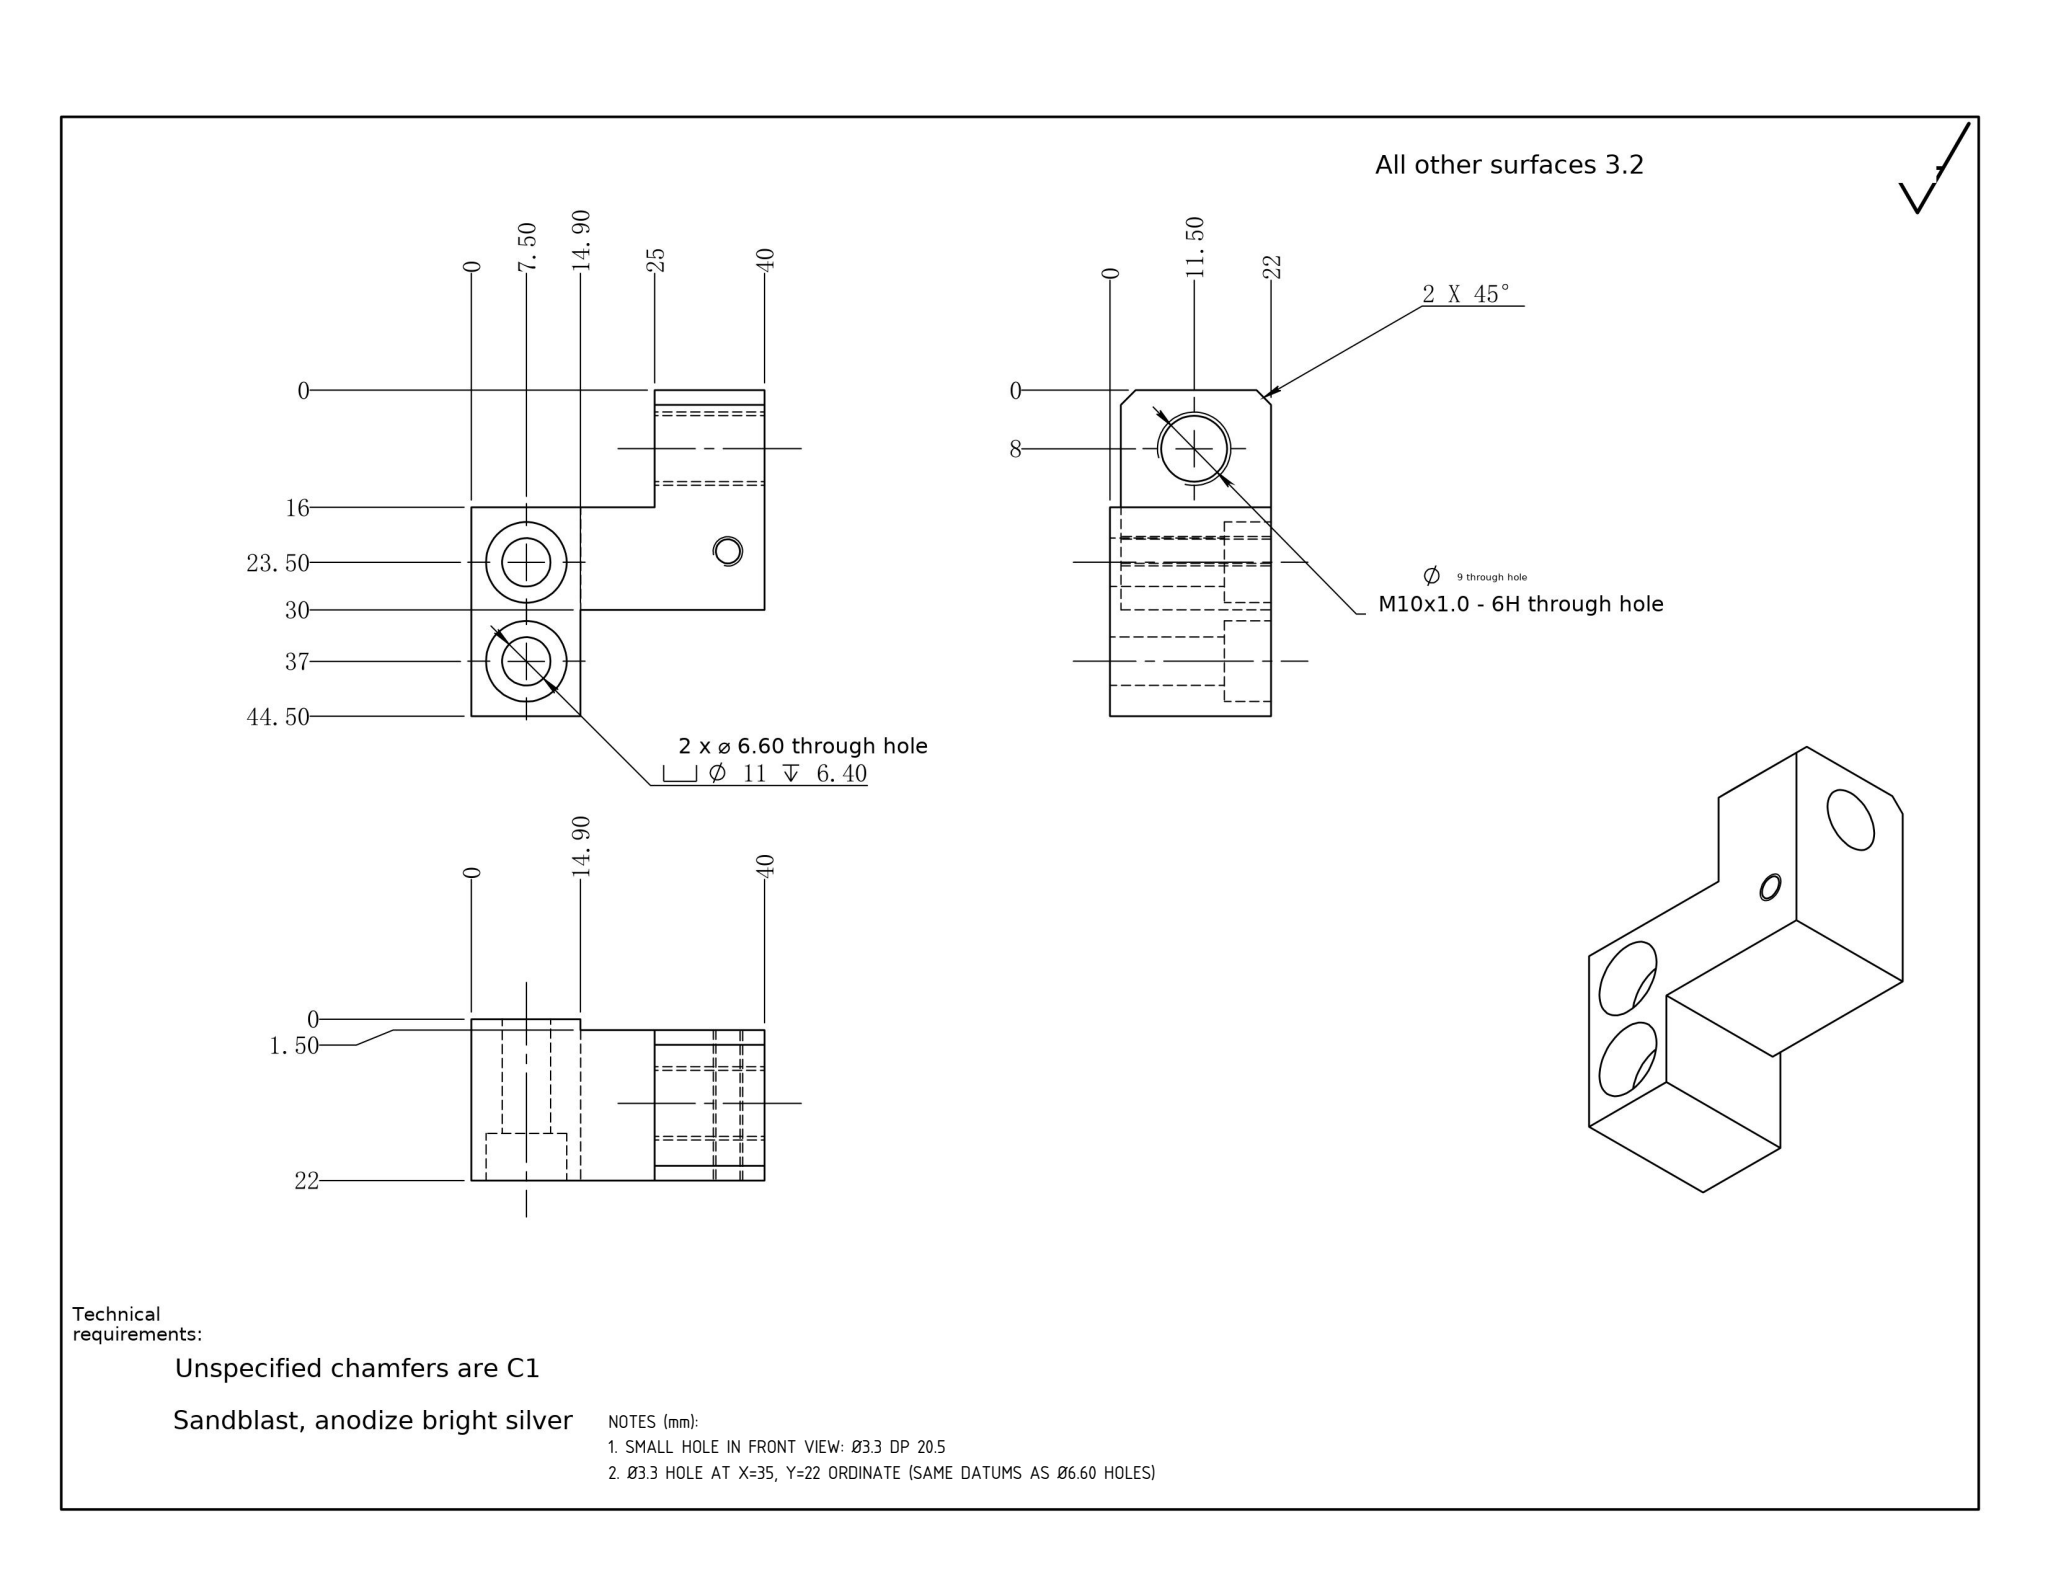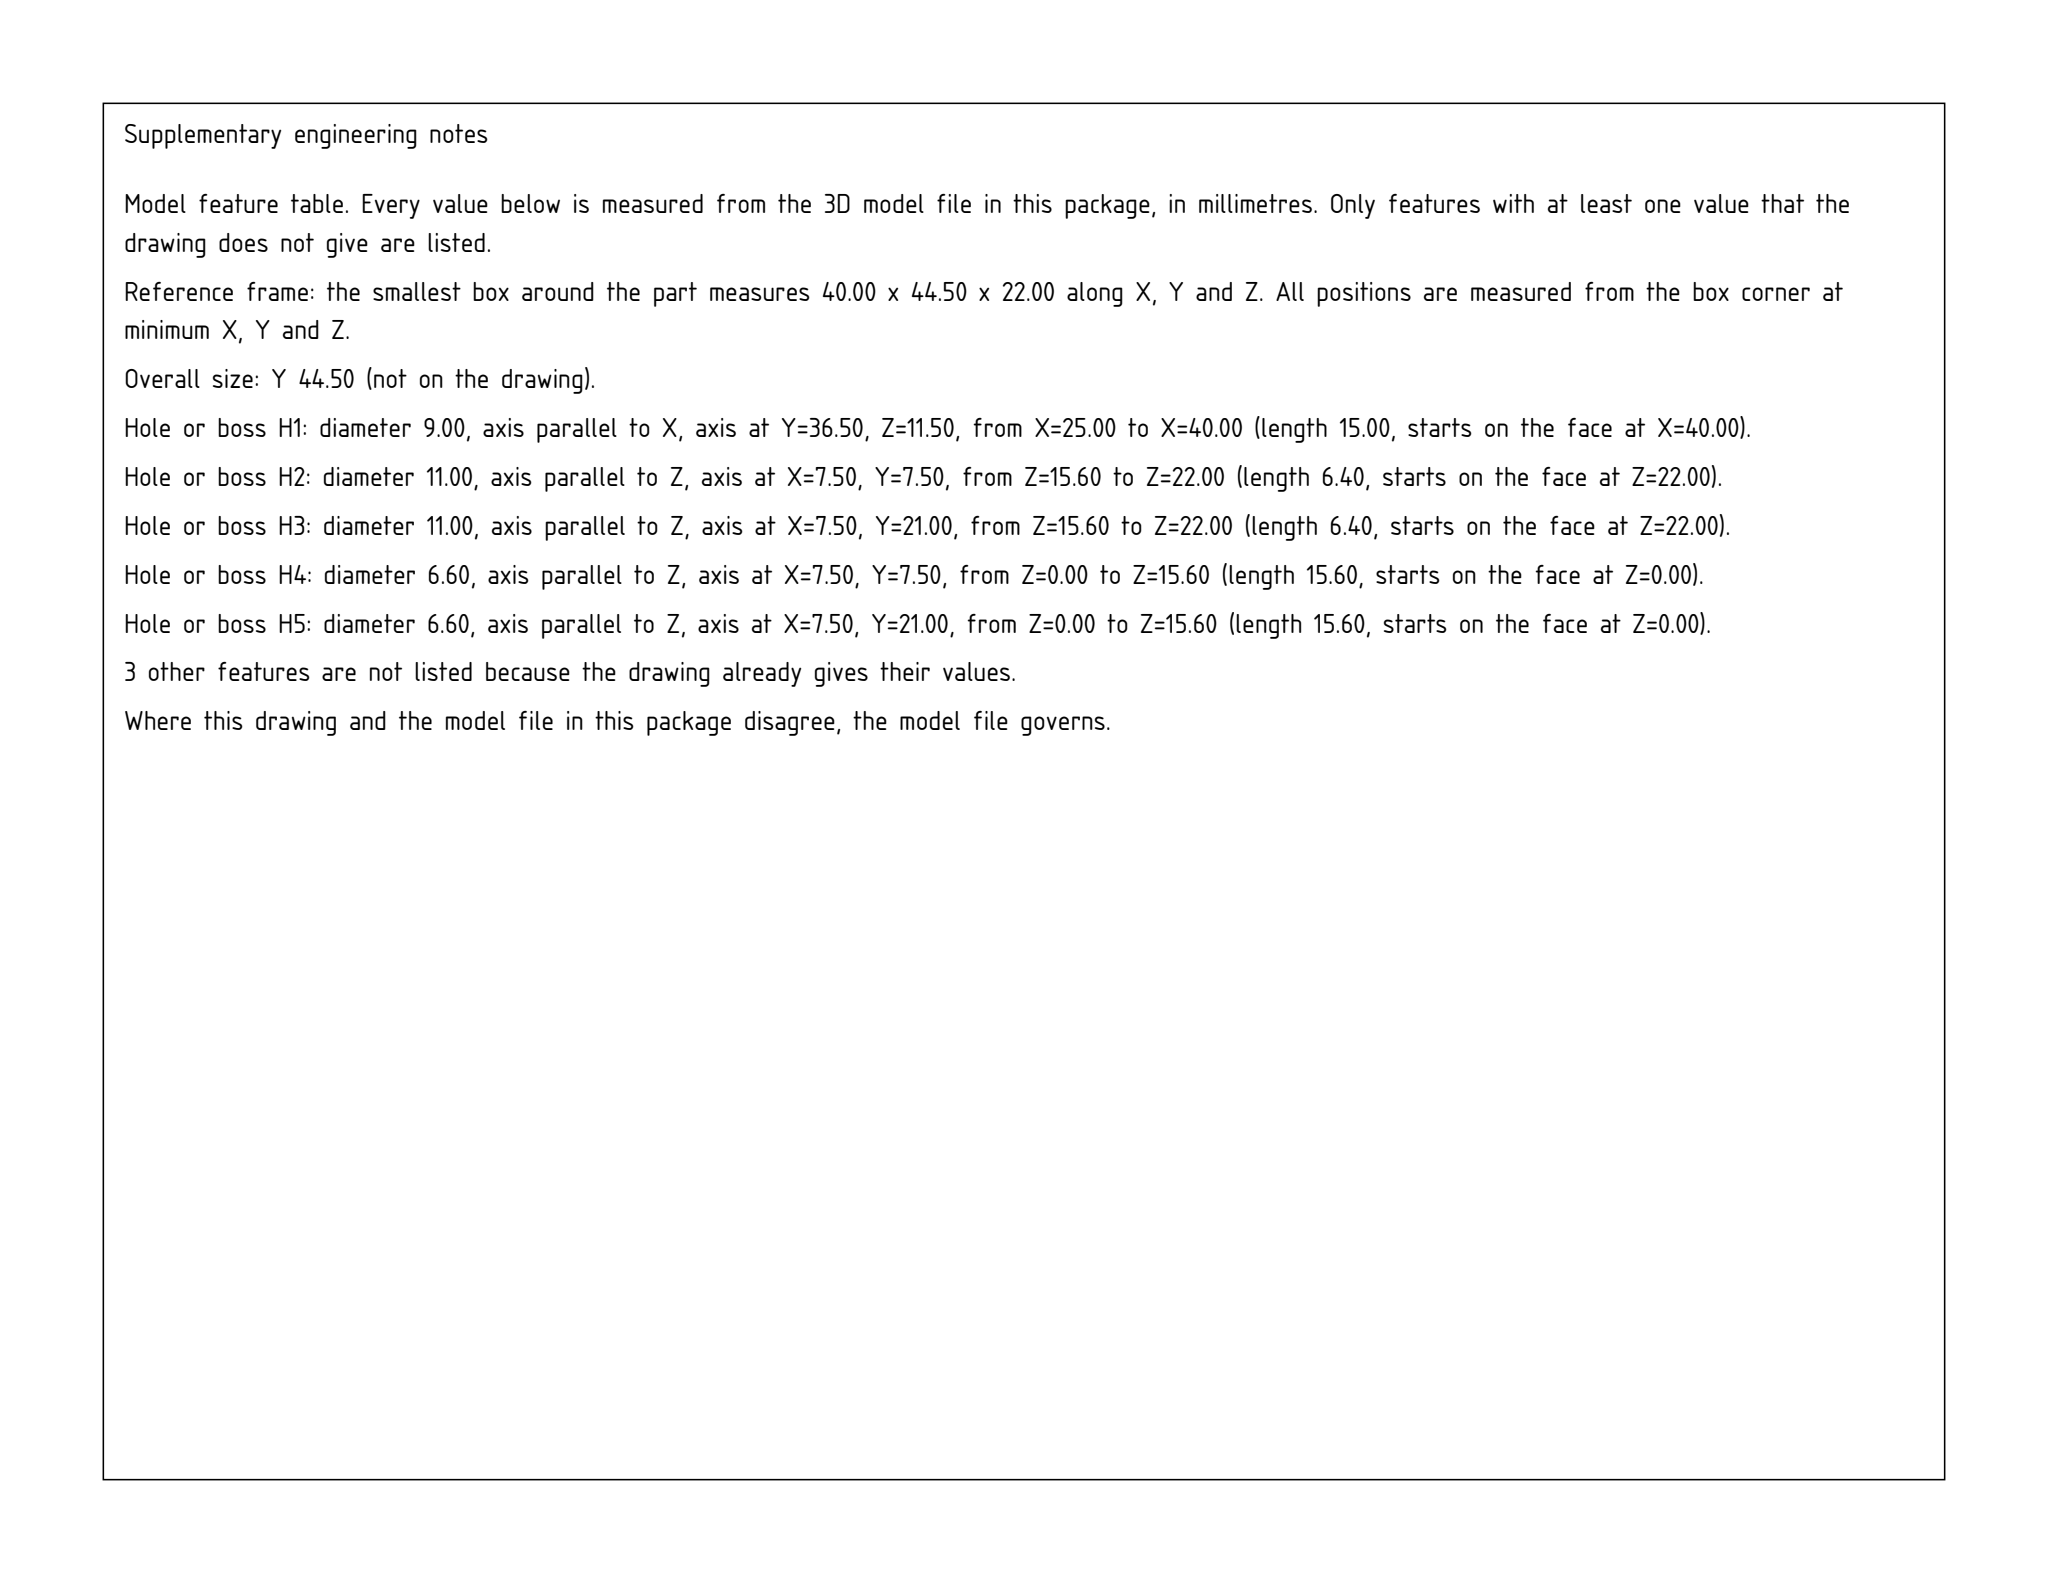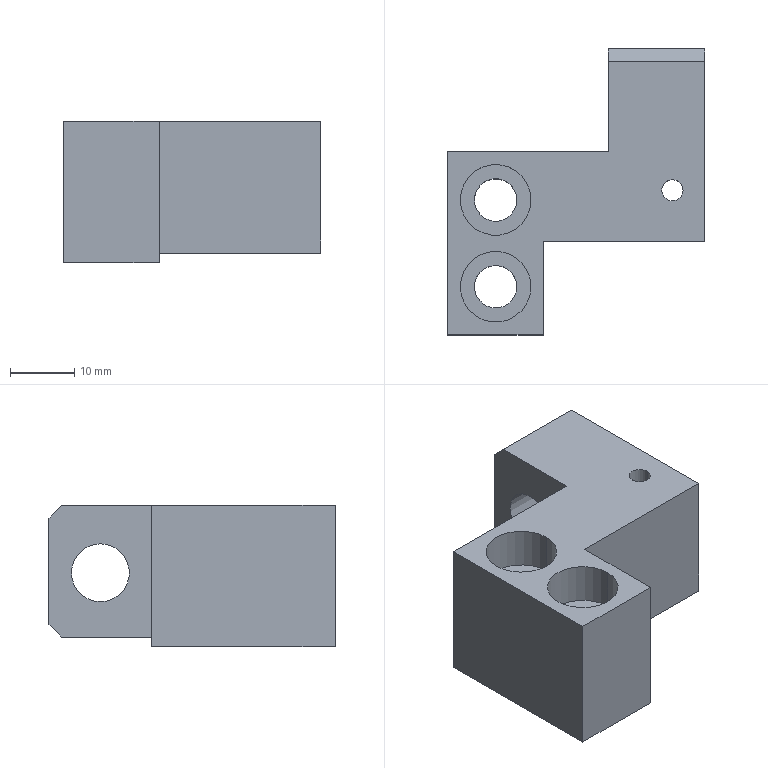Part | SolidWorks | mm | 1 solid | 27 faces | box 40 x 44.5 x 22 mm | volume 17993 mm3 | plane 15 | cylinder 12 | commonest cylinder face diameters 11 x4 6.6 x4 3.3 x2 9 x2
Drawing notes:
SMALL HOLE IN FRONT VIEW: Ø3.3 DP 20.5 | from the solid: cylinder dia 3.3, axis z, length 20.5 (blind, part 22 thick)
Ø3.3 HOLE AT X=35, Y=22 ORDINATE (SAME DATUMS AS Ø6.60 HOLES) | from the solid: pos [35.0, 22.5]; Y ordinate = 44.5-22.5 = 22, matching chain where y=21->23.50, y=7.5->37
build123d program:
from build123d import *

# Parameters (mm, degrees)
SKETCH1_W                                       = 40
SKETCH1_H                                       = 44.5
BOSS_EXTRUDE1_DEPTH                             = 22
M6_HEX_SOCKET_HEAD_CAP_SCREW_CBORE2_D           = 6.6
M6_HEX_SOCKET_HEAD_CAP_SCREW_CBORE2_CBORE_D     = 11
M6_HEX_SOCKET_HEAD_CAP_SCREW_CBORE2_CBORE_DEPTH = 6.4
SKETCH10_W                                      = 25.1
SKETCH10_H                                      = 14.5
CUT_EXTRUDE4_DEPTH                              = 26
SKETCH11_W                                      = 25
SKETCH11_H                                      = 16
CUT_EXTRUDE5_DEPTH                              = 22
SKETCH12_W                                      = 25.1
SKETCH12_H                                      = 30
CUT_EXTRUDE6_DEPTH                              = 1.5
M10X1_0_TAPPED_HOLE1_D                          = 9
CHAMFER2_SIZE                                   = 2
M4_TAPPED_HOLE1_D                               = 3.3


with BuildPart() as part:
    # Sketch1 → Boss-Extrude1 (new body)
    with BuildSketch(Plane.XY):
        Rectangle(SKETCH1_W, SKETCH1_H)
    extrude(amount=BOSS_EXTRUDE1_DEPTH)

    # M6 Hex Socket Head Cap Screw CBORE2 (through all)
    with Locations(Plane.XY.offset(22)):
        with Locations((-12.5, -1.25), (-12.5, -14.75)):
            CounterBoreHole(M6_HEX_SOCKET_HEAD_CAP_SCREW_CBORE2_D / 2, M6_HEX_SOCKET_HEAD_CAP_SCREW_CBORE2_CBORE_D / 2, M6_HEX_SOCKET_HEAD_CAP_SCREW_CBORE2_CBORE_DEPTH)

    # Sketch10 → Cut-Extrude4 (cut)
    with BuildSketch(Plane.XY.offset(22)):
        with Locations((7.45, -15)):
            Rectangle(SKETCH10_W, SKETCH10_H)
    extrude(amount=-CUT_EXTRUDE4_DEPTH, mode=Mode.SUBTRACT)

    # Sketch11 → Cut-Extrude5 (cut)
    with BuildSketch(Plane.XY.offset(22)):
        with Locations((-7.5, 14.25)):
            Rectangle(SKETCH11_W, SKETCH11_H)
    extrude(amount=-CUT_EXTRUDE5_DEPTH, mode=Mode.SUBTRACT)

    # Sketch12 → Cut-Extrude6 (cut)
    with BuildSketch(Plane(origin=(0, 0, 0), x_dir=(-1, 0, 0), z_dir=(0, 0, -1))):
        with Locations((-7.45, 7.25)):
            Rectangle(SKETCH12_W, SKETCH12_H)
    extrude(amount=-CUT_EXTRUDE6_DEPTH, mode=Mode.SUBTRACT)

    # M10x1.0 Tapped Hole1 (through all)
    with Locations(Plane.ZY.offset(-5)):
        with Locations((11.5, 14.25)):
            Hole(M10X1_0_TAPPED_HOLE1_D / 2)

    # Chamfer2
    chamfer2_edges = [part.edges().sort_by_distance(p)[0] for p in [
        (12.5, 22.25, 1.5),
        (12.5, 22.25, 22),
    ]]
    chamfer(chamfer2_edges, length=CHAMFER2_SIZE)

    # M4 Tapped Hole1 (through all)
    with Locations(Plane.XY.offset(22)):
        with Locations((15, 0.25)):
            Hole(M4_TAPPED_HOLE1_D / 2)


solid = part.part
STEP:
#1=CARTESIAN_POINT('',(16.65,0.25,1.5));
#2=VERTEX_POINT('',#1);
#3=CARTESIAN_POINT('',(13.35,0.25,1.5));
#4=VERTEX_POINT('',#3);
#5=CARTESIAN_POINT('',(15.,0.25,1.5));
#6=DIRECTION('',(0.,0.,-1.));
#7=DIRECTION('',(-1.,0.,0.));
#8=AXIS2_PLACEMENT_3D('',#5,#6,#7);
#9=CIRCLE('',#8,1.65);
#10=EDGE_CURVE('',#2,#4,#9,.T.);
#11=ORIENTED_EDGE('',*,*,#10,.T.);
#12=CARTESIAN_POINT('',(13.35,0.25,22.));
#13=VERTEX_POINT('',#12);
#14=CARTESIAN_POINT('',(13.35,0.25,22.));
#15=DIRECTION('',(0.,0.,1.));
#16=VECTOR('',#15,1000.);
#17=LINE('',#14,#16);
#18=EDGE_CURVE('',#4,#13,#17,.T.);
#19=ORIENTED_EDGE('',*,*,#18,.T.);
#20=CARTESIAN_POINT('',(16.65,0.25,22.));
#21=VERTEX_POINT('',#20);
#22=CARTESIAN_POINT('',(15.,0.25,22.));
#23=DIRECTION('',(0.,0.,1.));
#24=DIRECTION('',(1.,0.,0.));
#25=AXIS2_PLACEMENT_3D('',#22,#23,#24);
#26=CIRCLE('',#25,1.65);
#27=EDGE_CURVE('',#13,#21,#26,.T.);
#28=ORIENTED_EDGE('',*,*,#27,.T.);
#29=CARTESIAN_POINT('',(16.65,0.25,22.));
#30=DIRECTION('',(0.,0.,1.));
#31=VECTOR('',#30,1000.);
#32=LINE('',#29,#31);
#33=EDGE_CURVE('',#2,#21,#32,.T.);
#34=ORIENTED_EDGE('',*,*,#33,.F.);
#35=EDGE_LOOP('',(#11,#19,#28,#34));
#36=FACE_OUTER_BOUND('',#35,.T.);
#37=CARTESIAN_POINT('',(15.,0.25,22.));
#38=DIRECTION('',(0.,0.,1.));
#39=DIRECTION('',(1.,0.,0.));
#40=AXIS2_PLACEMENT_3D('',#37,#38,#39);
#41=CYLINDRICAL_SURFACE('',#40,1.65);
#42=ADVANCED_FACE('',(#36),#41,.F.);
#43=CARTESIAN_POINT('',(20.,14.25,7.));
#44=VERTEX_POINT('',#43);
#45=CARTESIAN_POINT('',(20.,14.25,16.));
#46=VERTEX_POINT('',#45);
#47=CARTESIAN_POINT('',(20.,14.25,11.5));
#48=DIRECTION('',(-1.,0.,0.));
#49=DIRECTION('',(0.,0.,1.));
#50=AXIS2_PLACEMENT_3D('',#47,#48,#49);
#51=CIRCLE('',#50,4.5);
#52=EDGE_CURVE('',#44,#46,#51,.T.);
#53=ORIENTED_EDGE('',*,*,#52,.F.);
#54=CARTESIAN_POINT('',(5.,14.25,7.));
#55=VERTEX_POINT('',#54);
#56=CARTESIAN_POINT('',(5.,14.25,7.));
#57=DIRECTION('',(-1.,0.,0.));
#58=VECTOR('',#57,1000.);
#59=LINE('',#56,#58);
#60=EDGE_CURVE('',#44,#55,#59,.T.);
#61=ORIENTED_EDGE('',*,*,#60,.T.);
#62=CARTESIAN_POINT('',(5.,14.25,16.));
#63=VERTEX_POINT('',#62);
#64=CARTESIAN_POINT('',(5.,14.25,11.5));
#65=DIRECTION('',(-1.,0.,0.));
#66=DIRECTION('',(0.,0.,1.));
#67=AXIS2_PLACEMENT_3D('',#64,#65,#66);
#68=CIRCLE('',#67,4.5);
#69=EDGE_CURVE('',#55,#63,#68,.T.);
#70=ORIENTED_EDGE('',*,*,#69,.T.);
#71=CARTESIAN_POINT('',(5.,14.25,16.));
#72=DIRECTION('',(-1.,0.,0.));
#73=VECTOR('',#72,1000.);
#74=LINE('',#71,#73);
#75=EDGE_CURVE('',#46,#63,#74,.T.);
#76=ORIENTED_EDGE('',*,*,#75,.F.);
#77=EDGE_LOOP('',(#53,#61,#70,#76));
#78=FACE_OUTER_BOUND('',#77,.T.);
#79=CARTESIAN_POINT('',(5.,14.25,11.5));
#80=DIRECTION('',(-1.,0.,0.));
#81=DIRECTION('',(0.,0.,1.));
#82=AXIS2_PLACEMENT_3D('',#79,#80,#81);
#83=CYLINDRICAL_SURFACE('',#82,4.5);
#84=ADVANCED_FACE('',(#78),#83,.F.);
#85=CARTESIAN_POINT('',(-18.,-1.25,15.6));
#86=VERTEX_POINT('',#85);
#87=CARTESIAN_POINT('',(-7.,-1.25,15.6));
#88=VERTEX_POINT('',#87);
#89=CARTESIAN_POINT('',(-12.5,-1.25,15.6));
#90=DIRECTION('',(0.,0.,1.));
#91=DIRECTION('',(1.,0.,0.));
#92=AXIS2_PLACEMENT_3D('',#89,#90,#91);
#93=CIRCLE('',#92,5.5);
#94=EDGE_CURVE('',#86,#88,#93,.T.);
#95=ORIENTED_EDGE('',*,*,#94,.F.);
#96=CARTESIAN_POINT('',(-18.,-1.25,22.));
#97=VERTEX_POINT('',#96);
#98=CARTESIAN_POINT('',(-18.,-1.25,22.));
#99=DIRECTION('',(0.,0.,1.));
#100=VECTOR('',#99,1000.);
#101=LINE('',#98,#100);
#102=EDGE_CURVE('',#86,#97,#101,.T.);
#103=ORIENTED_EDGE('',*,*,#102,.T.);
#104=CARTESIAN_POINT('',(-7.,-1.25,22.));
#105=VERTEX_POINT('',#104);
#106=CARTESIAN_POINT('',(-12.5,-1.25,22.));
#107=DIRECTION('',(0.,0.,1.));
#108=DIRECTION('',(1.,0.,0.));
#109=AXIS2_PLACEMENT_3D('',#106,#107,#108);
#110=CIRCLE('',#109,5.5);
#111=EDGE_CURVE('',#97,#105,#110,.T.);
#112=ORIENTED_EDGE('',*,*,#111,.T.);
#113=CARTESIAN_POINT('',(-7.,-1.25,22.));
#114=DIRECTION('',(0.,0.,1.));
#115=VECTOR('',#114,1000.);
#116=LINE('',#113,#115);
#117=EDGE_CURVE('',#88,#105,#116,.T.);
#118=ORIENTED_EDGE('',*,*,#117,.F.);
#119=EDGE_LOOP('',(#95,#103,#112,#118));
#120=FACE_OUTER_BOUND('',#119,.T.);
#121=CARTESIAN_POINT('',(-12.5,-1.25,22.));
#122=DIRECTION('',(0.,0.,1.));
#123=DIRECTION('',(1.,0.,0.));
#124=AXIS2_PLACEMENT_3D('',#121,#122,#123);
#125=CYLINDRICAL_SURFACE('',#124,5.5);
#126=ADVANCED_FACE('',(#120),#125,.F.);
#127=CARTESIAN_POINT('',(-15.8,-1.25,0.));
#128=VERTEX_POINT('',#127);
#129=CARTESIAN_POINT('',(-9.2,-1.25,0.));
#130=VERTEX_POINT('',#129);
#131=CARTESIAN_POINT('',(-12.5,-1.25,0.));
#132=DIRECTION('',(0.,0.,1.));
#133=DIRECTION('',(1.,0.,0.));
#134=AXIS2_PLACEMENT_3D('',#131,#132,#133);
#135=CIRCLE('',#134,3.3);
#136=EDGE_CURVE('',#128,#130,#135,.T.);
#137=ORIENTED_EDGE('',*,*,#136,.F.);
#138=CARTESIAN_POINT('',(-15.8,-1.25,15.6));
#139=VERTEX_POINT('',#138);
#140=CARTESIAN_POINT('',(-15.8,-1.25,22.));
#141=DIRECTION('',(0.,0.,1.));
#142=VECTOR('',#141,1000.);
#143=LINE('',#140,#142);
#144=EDGE_CURVE('',#128,#139,#143,.T.);
#145=ORIENTED_EDGE('',*,*,#144,.T.);
#146=CARTESIAN_POINT('',(-9.2,-1.25,15.6));
#147=VERTEX_POINT('',#146);
#148=CARTESIAN_POINT('',(-12.5,-1.25,15.6));
#149=DIRECTION('',(0.,0.,1.));
#150=DIRECTION('',(1.,0.,0.));
#151=AXIS2_PLACEMENT_3D('',#148,#149,#150);
#152=CIRCLE('',#151,3.3);
#153=EDGE_CURVE('',#139,#147,#152,.T.);
#154=ORIENTED_EDGE('',*,*,#153,.T.);
#155=CARTESIAN_POINT('',(-9.2,-1.25,22.));
#156=DIRECTION('',(0.,0.,1.));
#157=VECTOR('',#156,1000.);
#158=LINE('',#155,#157);
#159=EDGE_CURVE('',#130,#147,#158,.T.);
#160=ORIENTED_EDGE('',*,*,#159,.F.);
#161=EDGE_LOOP('',(#137,#145,#154,#160));
#162=FACE_OUTER_BOUND('',#161,.T.);
#163=CARTESIAN_POINT('',(-12.5,-1.25,22.));
#164=DIRECTION('',(0.,0.,1.));
#165=DIRECTION('',(1.,0.,0.));
#166=AXIS2_PLACEMENT_3D('',#163,#164,#165);
#167=CYLINDRICAL_SURFACE('',#166,3.3);
#168=ADVANCED_FACE('',(#162),#167,.F.);
#169=CARTESIAN_POINT('',(-18.,-14.75,15.6));
#170=VERTEX_POINT('',#169);
#171=CARTESIAN_POINT('',(-7.,-14.75,15.6));
#172=VERTEX_POINT('',#171);
#173=CARTESIAN_POINT('',(-12.5,-14.75,15.6));
#174=DIRECTION('',(0.,0.,1.));
#175=DIRECTION('',(1.,0.,0.));
#176=AXIS2_PLACEMENT_3D('',#173,#174,#175);
#177=CIRCLE('',#176,5.5);
#178=EDGE_CURVE('',#170,#172,#177,.T.);
#179=ORIENTED_EDGE('',*,*,#178,.F.);
#180=CARTESIAN_POINT('',(-18.,-14.75,22.));
#181=VERTEX_POINT('',#180);
#182=CARTESIAN_POINT('',(-18.,-14.75,22.));
#183=DIRECTION('',(0.,0.,1.));
#184=VECTOR('',#183,1000.);
#185=LINE('',#182,#184);
#186=EDGE_CURVE('',#170,#181,#185,.T.);
#187=ORIENTED_EDGE('',*,*,#186,.T.);
#188=CARTESIAN_POINT('',(-7.,-14.75,22.));
#189=VERTEX_POINT('',#188);
#190=CARTESIAN_POINT('',(-12.5,-14.75,22.));
#191=DIRECTION('',(0.,0.,1.));
#192=DIRECTION('',(1.,0.,0.));
#193=AXIS2_PLACEMENT_3D('',#190,#191,#192);
#194=CIRCLE('',#193,5.5);
#195=EDGE_CURVE('',#181,#189,#194,.T.);
#196=ORIENTED_EDGE('',*,*,#195,.T.);
#197=CARTESIAN_POINT('',(-7.,-14.75,22.));
#198=DIRECTION('',(0.,0.,1.));
#199=VECTOR('',#198,1000.);
#200=LINE('',#197,#199);
#201=EDGE_CURVE('',#172,#189,#200,.T.);
#202=ORIENTED_EDGE('',*,*,#201,.F.);
#203=EDGE_LOOP('',(#179,#187,#196,#202));
#204=FACE_OUTER_BOUND('',#203,.T.);
#205=CARTESIAN_POINT('',(-12.5,-14.75,22.));
#206=DIRECTION('',(0.,0.,1.));
#207=DIRECTION('',(1.,0.,0.));
#208=AXIS2_PLACEMENT_3D('',#205,#206,#207);
#209=CYLINDRICAL_SURFACE('',#208,5.5);
#210=ADVANCED_FACE('',(#204),#209,.F.);
#211=CARTESIAN_POINT('',(-15.8,-14.75,0.));
#212=VERTEX_POINT('',#211);
#213=CARTESIAN_POINT('',(-9.2,-14.75,0.));
#214=VERTEX_POINT('',#213);
#215=CARTESIAN_POINT('',(-12.5,-14.75,0.));
#216=DIRECTION('',(0.,0.,1.));
#217=DIRECTION('',(1.,0.,0.));
#218=AXIS2_PLACEMENT_3D('',#215,#216,#217);
#219=CIRCLE('',#218,3.3);
#220=EDGE_CURVE('',#212,#214,#219,.T.);
#221=ORIENTED_EDGE('',*,*,#220,.F.);
#222=CARTESIAN_POINT('',(-15.8,-14.75,15.6));
#223=VERTEX_POINT('',#222);
#224=CARTESIAN_POINT('',(-15.8,-14.75,22.));
#225=DIRECTION('',(0.,0.,1.));
#226=VECTOR('',#225,1000.);
#227=LINE('',#224,#226);
#228=EDGE_CURVE('',#212,#223,#227,.T.);
#229=ORIENTED_EDGE('',*,*,#228,.T.);
#230=CARTESIAN_POINT('',(-9.2,-14.75,15.6));
#231=VERTEX_POINT('',#230);
#232=CARTESIAN_POINT('',(-12.5,-14.75,15.6));
#233=DIRECTION('',(0.,0.,1.));
#234=DIRECTION('',(1.,0.,0.));
#235=AXIS2_PLACEMENT_3D('',#232,#233,#234);
#236=CIRCLE('',#235,3.3);
#237=EDGE_CURVE('',#223,#231,#236,.T.);
#238=ORIENTED_EDGE('',*,*,#237,.T.);
#239=CARTESIAN_POINT('',(-9.2,-14.75,22.));
#240=DIRECTION('',(0.,0.,1.));
#241=VECTOR('',#240,1000.);
#242=LINE('',#239,#241);
#243=EDGE_CURVE('',#214,#231,#242,.T.);
#244=ORIENTED_EDGE('',*,*,#243,.F.);
#245=EDGE_LOOP('',(#221,#229,#238,#244));
#246=FACE_OUTER_BOUND('',#245,.T.);
#247=CARTESIAN_POINT('',(-12.5,-14.75,22.));
#248=DIRECTION('',(0.,0.,1.));
#249=DIRECTION('',(1.,0.,0.));
#250=AXIS2_PLACEMENT_3D('',#247,#248,#249);
#251=CYLINDRICAL_SURFACE('',#250,3.3);
#252=ADVANCED_FACE('',(#246),#251,.F.);
#253=CARTESIAN_POINT('',(20.,14.25,11.5));
#254=DIRECTION('',(-1.,0.,0.));
#255=DIRECTION('',(0.,0.,1.));
#256=AXIS2_PLACEMENT_3D('',#253,#254,#255);
#257=CIRCLE('',#256,4.5);
#258=EDGE_CURVE('',#46,#44,#257,.T.);
#259=ORIENTED_EDGE('',*,*,#258,.T.);
#260=ORIENTED_EDGE('',*,*,#52,.T.);
#261=EDGE_LOOP('',(#259,#260));
#262=FACE_BOUND('',#261,.T.);
#263=CARTESIAN_POINT('',(20.,20.25,1.5));
#264=VERTEX_POINT('',#263);
#265=CARTESIAN_POINT('',(20.,-7.75,1.5));
#266=VERTEX_POINT('',#265);
#267=CARTESIAN_POINT('',(20.,22.25,1.5));
#268=DIRECTION('',(-0.,-1.,0.));
#269=VECTOR('',#268,1000.);
#270=LINE('',#267,#269);
#271=EDGE_CURVE('',#264,#266,#270,.T.);
#272=ORIENTED_EDGE('',*,*,#271,.F.);
#273=CARTESIAN_POINT('',(20.,22.25,3.5));
#274=VERTEX_POINT('',#273);
#275=CARTESIAN_POINT('',(20.,20.25,1.5));
#276=DIRECTION('',(0.,0.7071,0.7071));
#277=VECTOR('',#276,1000.);
#278=LINE('',#275,#277);
#279=EDGE_CURVE('',#264,#274,#278,.T.);
#280=ORIENTED_EDGE('',*,*,#279,.T.);
#281=CARTESIAN_POINT('',(20.,22.25,20.));
#282=VERTEX_POINT('',#281);
#283=CARTESIAN_POINT('',(20.,22.25,22.));
#284=DIRECTION('',(0.,0.,-1.));
#285=VECTOR('',#284,1000.);
#286=LINE('',#283,#285);
#287=EDGE_CURVE('',#282,#274,#286,.T.);
#288=ORIENTED_EDGE('',*,*,#287,.F.);
#289=CARTESIAN_POINT('',(20.,20.25,22.));
#290=VERTEX_POINT('',#289);
#291=CARTESIAN_POINT('',(20.,20.25,22.));
#292=DIRECTION('',(0.,-0.7071,0.7071));
#293=VECTOR('',#292,1000.);
#294=LINE('',#291,#293);
#295=EDGE_CURVE('',#282,#290,#294,.T.);
#296=ORIENTED_EDGE('',*,*,#295,.T.);
#297=CARTESIAN_POINT('',(20.,-7.75,22.));
#298=VERTEX_POINT('',#297);
#299=CARTESIAN_POINT('',(20.,-22.25,22.));
#300=DIRECTION('',(0.,1.,0.));
#301=VECTOR('',#300,1000.);
#302=LINE('',#299,#301);
#303=EDGE_CURVE('',#298,#290,#302,.T.);
#304=ORIENTED_EDGE('',*,*,#303,.F.);
#305=CARTESIAN_POINT('',(20.,-7.75,-4.));
#306=DIRECTION('',(0.,0.,1.));
#307=VECTOR('',#306,1000.);
#308=LINE('',#305,#307);
#309=EDGE_CURVE('',#266,#298,#308,.T.);
#310=ORIENTED_EDGE('',*,*,#309,.F.);
#311=EDGE_LOOP('',(#272,#280,#288,#296,#304,#310));
#312=FACE_OUTER_BOUND('',#311,.T.);
#313=CARTESIAN_POINT('',(20.,-22.25,22.));
#314=DIRECTION('',(-1.,0.,0.));
#315=DIRECTION('',(0.,0.,1.));
#316=AXIS2_PLACEMENT_3D('',#313,#314,#315);
#317=PLANE('',#316);
#318=ADVANCED_FACE('',(#262,#312),#317,.F.);
#319=ORIENTED_EDGE('',*,*,#287,.T.);
#320=CARTESIAN_POINT('',(5.,22.25,3.5));
#321=VERTEX_POINT('',#320);
#322=CARTESIAN_POINT('',(5.,22.25,3.5));
#323=DIRECTION('',(-1.,0.,0.));
#324=VECTOR('',#323,1000.);
#325=LINE('',#322,#324);
#326=EDGE_CURVE('',#274,#321,#325,.T.);
#327=ORIENTED_EDGE('',*,*,#326,.T.);
#328=CARTESIAN_POINT('',(5.,22.25,20.));
#329=VERTEX_POINT('',#328);
#330=CARTESIAN_POINT('',(5.,22.25,0.));
#331=DIRECTION('',(0.,0.,1.));
#332=VECTOR('',#331,1000.);
#333=LINE('',#330,#332);
#334=EDGE_CURVE('',#321,#329,#333,.T.);
#335=ORIENTED_EDGE('',*,*,#334,.T.);
#336=CARTESIAN_POINT('',(-20.,22.25,20.));
#337=DIRECTION('',(1.,0.,0.));
#338=VECTOR('',#337,1000.);
#339=LINE('',#336,#338);
#340=EDGE_CURVE('',#329,#282,#339,.T.);
#341=ORIENTED_EDGE('',*,*,#340,.T.);
#342=EDGE_LOOP('',(#319,#327,#335,#341));
#343=FACE_OUTER_BOUND('',#342,.T.);
#344=CARTESIAN_POINT('',(-20.,22.25,22.));
#345=DIRECTION('',(0.,-1.,0.));
#346=DIRECTION('',(0.,0.,-1.));
#347=AXIS2_PLACEMENT_3D('',#344,#345,#346);
#348=PLANE('',#347);
#349=ADVANCED_FACE('',(#343),#348,.F.);
#350=CARTESIAN_POINT('',(-5.1,-7.75,1.5));
#351=VERTEX_POINT('',#350);
#352=CARTESIAN_POINT('',(20.,-7.75,1.5));
#353=DIRECTION('',(-1.,0.,0.));
#354=VECTOR('',#353,1000.);
#355=LINE('',#352,#354);
#356=EDGE_CURVE('',#266,#351,#355,.T.);
#357=ORIENTED_EDGE('',*,*,#356,.F.);
#358=ORIENTED_EDGE('',*,*,#309,.T.);
#359=CARTESIAN_POINT('',(-5.1,-7.75,22.));
#360=VERTEX_POINT('',#359);
#361=CARTESIAN_POINT('',(20.,-7.75,22.));
#362=DIRECTION('',(-1.,-0.,0.));
#363=VECTOR('',#362,1000.);
#364=LINE('',#361,#363);
#365=EDGE_CURVE('',#298,#360,#364,.T.);
#366=ORIENTED_EDGE('',*,*,#365,.T.);
#367=CARTESIAN_POINT('',(-5.1,-7.75,-4.));
#368=DIRECTION('',(0.,0.,1.));
#369=VECTOR('',#368,1000.);
#370=LINE('',#367,#369);
#371=EDGE_CURVE('',#351,#360,#370,.T.);
#372=ORIENTED_EDGE('',*,*,#371,.F.);
#373=EDGE_LOOP('',(#357,#358,#366,#372));
#374=FACE_OUTER_BOUND('',#373,.T.);
#375=CARTESIAN_POINT('',(20.,-7.75,-4.));
#376=DIRECTION('',(-0.,1.,0.));
#377=DIRECTION('',(-1.,-0.,0.));
#378=AXIS2_PLACEMENT_3D('',#375,#376,#377);
#379=PLANE('',#378);
#380=ADVANCED_FACE('',(#374),#379,.F.);
#381=CARTESIAN_POINT('',(5.,14.25,11.5));
#382=DIRECTION('',(-1.,0.,0.));
#383=DIRECTION('',(0.,0.,1.));
#384=AXIS2_PLACEMENT_3D('',#381,#382,#383);
#385=CIRCLE('',#384,4.5);
#386=EDGE_CURVE('',#63,#55,#385,.T.);
#387=ORIENTED_EDGE('',*,*,#386,.F.);
#388=ORIENTED_EDGE('',*,*,#69,.F.);
#389=EDGE_LOOP('',(#387,#388));
#390=FACE_BOUND('',#389,.T.);
#391=ORIENTED_EDGE('',*,*,#334,.F.);
#392=CARTESIAN_POINT('',(5.,20.25,1.5));
#393=VERTEX_POINT('',#392);
#394=CARTESIAN_POINT('',(5.,20.25,1.5));
#395=DIRECTION('',(0.,-0.7071,-0.7071));
#396=VECTOR('',#395,1000.);
#397=LINE('',#394,#396);
#398=EDGE_CURVE('',#321,#393,#397,.T.);
#399=ORIENTED_EDGE('',*,*,#398,.T.);
#400=CARTESIAN_POINT('',(5.,6.25,1.5));
#401=VERTEX_POINT('',#400);
#402=CARTESIAN_POINT('',(5.,22.25,1.5));
#403=DIRECTION('',(-0.,1.,0.));
#404=VECTOR('',#403,1000.);
#405=LINE('',#402,#404);
#406=EDGE_CURVE('',#401,#393,#405,.T.);
#407=ORIENTED_EDGE('',*,*,#406,.F.);
#408=CARTESIAN_POINT('',(5.,6.25,22.));
#409=VERTEX_POINT('',#408);
#410=CARTESIAN_POINT('',(5.,6.25,0.));
#411=DIRECTION('',(0.,0.,1.));
#412=VECTOR('',#411,1000.);
#413=LINE('',#410,#412);
#414=EDGE_CURVE('',#401,#409,#413,.T.);
#415=ORIENTED_EDGE('',*,*,#414,.T.);
#416=CARTESIAN_POINT('',(5.,20.25,22.));
#417=VERTEX_POINT('',#416);
#418=CARTESIAN_POINT('',(5.,22.25,22.));
#419=DIRECTION('',(-0.,1.,0.));
#420=VECTOR('',#419,1000.);
#421=LINE('',#418,#420);
#422=EDGE_CURVE('',#409,#417,#421,.T.);
#423=ORIENTED_EDGE('',*,*,#422,.T.);
#424=CARTESIAN_POINT('',(5.,20.25,22.));
#425=DIRECTION('',(-0.,0.7071,-0.7071));
#426=VECTOR('',#425,1000.);
#427=LINE('',#424,#426);
#428=EDGE_CURVE('',#417,#329,#427,.T.);
#429=ORIENTED_EDGE('',*,*,#428,.T.);
#430=EDGE_LOOP('',(#391,#399,#407,#415,#423,#429));
#431=FACE_OUTER_BOUND('',#430,.T.);
#432=CARTESIAN_POINT('',(5.,22.25,0.));
#433=DIRECTION('',(1.,0.,0.));
#434=DIRECTION('',(-0.,1.,0.));
#435=AXIS2_PLACEMENT_3D('',#432,#433,#434);
#436=PLANE('',#435);
#437=ADVANCED_FACE('',(#390,#431),#436,.F.);
#438=CARTESIAN_POINT('',(-20.,6.25,22.));
#439=VERTEX_POINT('',#438);
#440=CARTESIAN_POINT('',(-20.,-22.25,22.));
#441=VERTEX_POINT('',#440);
#442=CARTESIAN_POINT('',(-20.,-22.25,22.));
#443=DIRECTION('',(0.,-1.,0.));
#444=VECTOR('',#443,1000.);
#445=LINE('',#442,#444);
#446=EDGE_CURVE('',#439,#441,#445,.T.);
#447=ORIENTED_EDGE('',*,*,#446,.F.);
#448=CARTESIAN_POINT('',(-20.,6.25,0.));
#449=VERTEX_POINT('',#448);
#450=CARTESIAN_POINT('',(-20.,6.25,0.));
#451=DIRECTION('',(0.,0.,1.));
#452=VECTOR('',#451,1000.);
#453=LINE('',#450,#452);
#454=EDGE_CURVE('',#449,#439,#453,.T.);
#455=ORIENTED_EDGE('',*,*,#454,.F.);
#456=CARTESIAN_POINT('',(-20.,-22.25,0.));
#457=VERTEX_POINT('',#456);
#458=CARTESIAN_POINT('',(-20.,-22.25,0.));
#459=DIRECTION('',(0.,-1.,0.));
#460=VECTOR('',#459,1000.);
#461=LINE('',#458,#460);
#462=EDGE_CURVE('',#449,#457,#461,.T.);
#463=ORIENTED_EDGE('',*,*,#462,.T.);
#464=CARTESIAN_POINT('',(-20.,-22.25,22.));
#465=DIRECTION('',(0.,0.,-1.));
#466=VECTOR('',#465,1000.);
#467=LINE('',#464,#466);
#468=EDGE_CURVE('',#441,#457,#467,.T.);
#469=ORIENTED_EDGE('',*,*,#468,.F.);
#470=EDGE_LOOP('',(#447,#455,#463,#469));
#471=FACE_OUTER_BOUND('',#470,.T.);
#472=CARTESIAN_POINT('',(-20.,-22.25,22.));
#473=DIRECTION('',(1.,0.,0.));
#474=DIRECTION('',(0.,0.,-1.));
#475=AXIS2_PLACEMENT_3D('',#472,#473,#474);
#476=PLANE('',#475);
#477=ADVANCED_FACE('',(#471),#476,.F.);
#478=CARTESIAN_POINT('',(-5.1,-22.25,-0.));
#479=VERTEX_POINT('',#478);
#480=CARTESIAN_POINT('',(-20.,-22.25,0.));
#481=DIRECTION('',(1.,0.,0.));
#482=VECTOR('',#481,1000.);
#483=LINE('',#480,#482);
#484=EDGE_CURVE('',#457,#479,#483,.T.);
#485=ORIENTED_EDGE('',*,*,#484,.T.);
#486=CARTESIAN_POINT('',(-5.1,-22.25,22.));
#487=VERTEX_POINT('',#486);
#488=CARTESIAN_POINT('',(-5.1,-22.25,-4.));
#489=DIRECTION('',(0.,0.,1.));
#490=VECTOR('',#489,1000.);
#491=LINE('',#488,#490);
#492=EDGE_CURVE('',#479,#487,#491,.T.);
#493=ORIENTED_EDGE('',*,*,#492,.T.);
#494=CARTESIAN_POINT('',(-20.,-22.25,22.));
#495=DIRECTION('',(1.,0.,0.));
#496=VECTOR('',#495,1000.);
#497=LINE('',#494,#496);
#498=EDGE_CURVE('',#441,#487,#497,.T.);
#499=ORIENTED_EDGE('',*,*,#498,.F.);
#500=ORIENTED_EDGE('',*,*,#468,.T.);
#501=EDGE_LOOP('',(#485,#493,#499,#500));
#502=FACE_OUTER_BOUND('',#501,.T.);
#503=CARTESIAN_POINT('',(-20.,-22.25,22.));
#504=DIRECTION('',(0.,1.,0.));
#505=DIRECTION('',(0.,0.,1.));
#506=AXIS2_PLACEMENT_3D('',#503,#504,#505);
#507=PLANE('',#506);
#508=ADVANCED_FACE('',(#502),#507,.F.);
#509=CARTESIAN_POINT('',(15.,0.25,22.));
#510=DIRECTION('',(0.,0.,1.));
#511=DIRECTION('',(1.,0.,0.));
#512=AXIS2_PLACEMENT_3D('',#509,#510,#511);
#513=CIRCLE('',#512,1.65);
#514=EDGE_CURVE('',#21,#13,#513,.T.);
#515=ORIENTED_EDGE('',*,*,#514,.F.);
#516=ORIENTED_EDGE('',*,*,#27,.F.);
#517=EDGE_LOOP('',(#515,#516));
#518=FACE_BOUND('',#517,.T.);
#519=CARTESIAN_POINT('',(-12.5,-1.25,22.));
#520=DIRECTION('',(0.,0.,1.));
#521=DIRECTION('',(1.,0.,0.));
#522=AXIS2_PLACEMENT_3D('',#519,#520,#521);
#523=CIRCLE('',#522,5.5);
#524=EDGE_CURVE('',#105,#97,#523,.T.);
#525=ORIENTED_EDGE('',*,*,#524,.F.);
#526=ORIENTED_EDGE('',*,*,#111,.F.);
#527=EDGE_LOOP('',(#525,#526));
#528=FACE_BOUND('',#527,.T.);
#529=CARTESIAN_POINT('',(-12.5,-14.75,22.));
#530=DIRECTION('',(0.,0.,1.));
#531=DIRECTION('',(1.,0.,0.));
#532=AXIS2_PLACEMENT_3D('',#529,#530,#531);
#533=CIRCLE('',#532,5.5);
#534=EDGE_CURVE('',#189,#181,#533,.T.);
#535=ORIENTED_EDGE('',*,*,#534,.F.);
#536=ORIENTED_EDGE('',*,*,#195,.F.);
#537=EDGE_LOOP('',(#535,#536));
#538=FACE_BOUND('',#537,.T.);
#539=ORIENTED_EDGE('',*,*,#303,.T.);
#540=CARTESIAN_POINT('',(0.,20.25,22.));
#541=DIRECTION('',(-1.,0.,0.));
#542=VECTOR('',#541,1000.);
#543=LINE('',#540,#542);
#544=EDGE_CURVE('',#290,#417,#543,.T.);
#545=ORIENTED_EDGE('',*,*,#544,.T.);
#546=ORIENTED_EDGE('',*,*,#422,.F.);
#547=CARTESIAN_POINT('',(-20.,6.25,22.));
#548=DIRECTION('',(1.,0.,0.));
#549=VECTOR('',#548,1000.);
#550=LINE('',#547,#549);
#551=EDGE_CURVE('',#439,#409,#550,.T.);
#552=ORIENTED_EDGE('',*,*,#551,.F.);
#553=ORIENTED_EDGE('',*,*,#446,.T.);
#554=ORIENTED_EDGE('',*,*,#498,.T.);
#555=CARTESIAN_POINT('',(-5.1,-22.25,22.));
#556=DIRECTION('',(0.,-1.,0.));
#557=VECTOR('',#556,1000.);
#558=LINE('',#555,#557);
#559=EDGE_CURVE('',#360,#487,#558,.T.);
#560=ORIENTED_EDGE('',*,*,#559,.F.);
#561=ORIENTED_EDGE('',*,*,#365,.F.);
#562=EDGE_LOOP('',(#539,#545,#546,#552,#553,#554,#560,#561));
#563=FACE_OUTER_BOUND('',#562,.T.);
#564=CARTESIAN_POINT('',(0.,0.,22.));
#565=DIRECTION('',(0.,0.,-1.));
#566=DIRECTION('',(-1.,0.,0.));
#567=AXIS2_PLACEMENT_3D('',#564,#565,#566);
#568=PLANE('',#567);
#569=ADVANCED_FACE('',(#518,#528,#538,#563),#568,.F.);
#570=CARTESIAN_POINT('',(-5.1,6.25,0.));
#571=VERTEX_POINT('',#570);
#572=CARTESIAN_POINT('',(-20.,6.25,0.));
#573=DIRECTION('',(1.,0.,0.));
#574=VECTOR('',#573,1000.);
#575=LINE('',#572,#574);
#576=EDGE_CURVE('',#449,#571,#575,.T.);
#577=ORIENTED_EDGE('',*,*,#576,.T.);
#578=CARTESIAN_POINT('',(-5.1,0.,0.));
#579=DIRECTION('',(0.,1.,0.));
#580=VECTOR('',#579,1000.);
#581=LINE('',#578,#580);
#582=EDGE_CURVE('',#479,#571,#581,.T.);
#583=ORIENTED_EDGE('',*,*,#582,.F.);
#584=ORIENTED_EDGE('',*,*,#484,.F.);
#585=ORIENTED_EDGE('',*,*,#462,.F.);
#586=EDGE_LOOP('',(#577,#583,#584,#585));
#587=FACE_OUTER_BOUND('',#586,.T.);
#588=CARTESIAN_POINT('',(-12.5,-1.25,0.));
#589=DIRECTION('',(0.,0.,1.));
#590=DIRECTION('',(1.,0.,0.));
#591=AXIS2_PLACEMENT_3D('',#588,#589,#590);
#592=CIRCLE('',#591,3.3);
#593=EDGE_CURVE('',#130,#128,#592,.T.);
#594=ORIENTED_EDGE('',*,*,#593,.T.);
#595=ORIENTED_EDGE('',*,*,#136,.T.);
#596=EDGE_LOOP('',(#594,#595));
#597=FACE_BOUND('',#596,.T.);
#598=CARTESIAN_POINT('',(-12.5,-14.75,0.));
#599=DIRECTION('',(0.,0.,1.));
#600=DIRECTION('',(1.,0.,0.));
#601=AXIS2_PLACEMENT_3D('',#598,#599,#600);
#602=CIRCLE('',#601,3.3);
#603=EDGE_CURVE('',#214,#212,#602,.T.);
#604=ORIENTED_EDGE('',*,*,#603,.T.);
#605=ORIENTED_EDGE('',*,*,#220,.T.);
#606=EDGE_LOOP('',(#604,#605));
#607=FACE_BOUND('',#606,.T.);
#608=CARTESIAN_POINT('',(0.,0.,0.));
#609=DIRECTION('',(0.,0.,-1.));
#610=DIRECTION('',(-1.,0.,0.));
#611=AXIS2_PLACEMENT_3D('',#608,#609,#610);
#612=PLANE('',#611);
#613=ADVANCED_FACE('',(#587,#597,#607),#612,.T.);
#614=ORIENTED_EDGE('',*,*,#228,.F.);
#615=ORIENTED_EDGE('',*,*,#603,.F.);
#616=ORIENTED_EDGE('',*,*,#243,.T.);
#617=CARTESIAN_POINT('',(-12.5,-14.75,15.6));
#618=DIRECTION('',(0.,0.,1.));
#619=DIRECTION('',(1.,0.,0.));
#620=AXIS2_PLACEMENT_3D('',#617,#618,#619);
#621=CIRCLE('',#620,3.3);
#622=EDGE_CURVE('',#231,#223,#621,.T.);
#623=ORIENTED_EDGE('',*,*,#622,.T.);
#624=EDGE_LOOP('',(#614,#615,#616,#623));
#625=FACE_OUTER_BOUND('',#624,.T.);
#626=CARTESIAN_POINT('',(-12.5,-14.75,22.));
#627=DIRECTION('',(0.,0.,1.));
#628=DIRECTION('',(1.,0.,0.));
#629=AXIS2_PLACEMENT_3D('',#626,#627,#628);
#630=CYLINDRICAL_SURFACE('',#629,3.3);
#631=ADVANCED_FACE('',(#625),#630,.F.);
#632=ORIENTED_EDGE('',*,*,#622,.F.);
#633=ORIENTED_EDGE('',*,*,#237,.F.);
#634=EDGE_LOOP('',(#632,#633));
#635=FACE_BOUND('',#634,.T.);
#636=CARTESIAN_POINT('',(-12.5,-14.75,15.6));
#637=DIRECTION('',(0.,0.,1.));
#638=DIRECTION('',(1.,0.,0.));
#639=AXIS2_PLACEMENT_3D('',#636,#637,#638);
#640=CIRCLE('',#639,5.5);
#641=EDGE_CURVE('',#172,#170,#640,.T.);
#642=ORIENTED_EDGE('',*,*,#641,.T.);
#643=ORIENTED_EDGE('',*,*,#178,.T.);
#644=EDGE_LOOP('',(#642,#643));
#645=FACE_OUTER_BOUND('',#644,.T.);
#646=CARTESIAN_POINT('',(-9.2,-14.75,15.6));
#647=DIRECTION('',(0.,0.,-1.));
#648=DIRECTION('',(-1.,0.,0.));
#649=AXIS2_PLACEMENT_3D('',#646,#647,#648);
#650=PLANE('',#649);
#651=ADVANCED_FACE('',(#635,#645),#650,.F.);
#652=ORIENTED_EDGE('',*,*,#186,.F.);
#653=ORIENTED_EDGE('',*,*,#641,.F.);
#654=ORIENTED_EDGE('',*,*,#201,.T.);
#655=ORIENTED_EDGE('',*,*,#534,.T.);
#656=EDGE_LOOP('',(#652,#653,#654,#655));
#657=FACE_OUTER_BOUND('',#656,.T.);
#658=CARTESIAN_POINT('',(-12.5,-14.75,22.));
#659=DIRECTION('',(0.,0.,1.));
#660=DIRECTION('',(1.,0.,0.));
#661=AXIS2_PLACEMENT_3D('',#658,#659,#660);
#662=CYLINDRICAL_SURFACE('',#661,5.5);
#663=ADVANCED_FACE('',(#657),#662,.F.);
#664=ORIENTED_EDGE('',*,*,#144,.F.);
#665=ORIENTED_EDGE('',*,*,#593,.F.);
#666=ORIENTED_EDGE('',*,*,#159,.T.);
#667=CARTESIAN_POINT('',(-12.5,-1.25,15.6));
#668=DIRECTION('',(0.,0.,1.));
#669=DIRECTION('',(1.,0.,0.));
#670=AXIS2_PLACEMENT_3D('',#667,#668,#669);
#671=CIRCLE('',#670,3.3);
#672=EDGE_CURVE('',#147,#139,#671,.T.);
#673=ORIENTED_EDGE('',*,*,#672,.T.);
#674=EDGE_LOOP('',(#664,#665,#666,#673));
#675=FACE_OUTER_BOUND('',#674,.T.);
#676=CARTESIAN_POINT('',(-12.5,-1.25,22.));
#677=DIRECTION('',(0.,0.,1.));
#678=DIRECTION('',(1.,0.,0.));
#679=AXIS2_PLACEMENT_3D('',#676,#677,#678);
#680=CYLINDRICAL_SURFACE('',#679,3.3);
#681=ADVANCED_FACE('',(#675),#680,.F.);
#682=ORIENTED_EDGE('',*,*,#672,.F.);
#683=ORIENTED_EDGE('',*,*,#153,.F.);
#684=EDGE_LOOP('',(#682,#683));
#685=FACE_BOUND('',#684,.T.);
#686=CARTESIAN_POINT('',(-12.5,-1.25,15.6));
#687=DIRECTION('',(0.,0.,1.));
#688=DIRECTION('',(1.,0.,0.));
#689=AXIS2_PLACEMENT_3D('',#686,#687,#688);
#690=CIRCLE('',#689,5.5);
#691=EDGE_CURVE('',#88,#86,#690,.T.);
#692=ORIENTED_EDGE('',*,*,#691,.T.);
#693=ORIENTED_EDGE('',*,*,#94,.T.);
#694=EDGE_LOOP('',(#692,#693));
#695=FACE_OUTER_BOUND('',#694,.T.);
#696=CARTESIAN_POINT('',(-9.2,-1.25,15.6));
#697=DIRECTION('',(0.,0.,-1.));
#698=DIRECTION('',(-1.,0.,0.));
#699=AXIS2_PLACEMENT_3D('',#696,#697,#698);
#700=PLANE('',#699);
#701=ADVANCED_FACE('',(#685,#695),#700,.F.);
#702=ORIENTED_EDGE('',*,*,#102,.F.);
#703=ORIENTED_EDGE('',*,*,#691,.F.);
#704=ORIENTED_EDGE('',*,*,#117,.T.);
#705=ORIENTED_EDGE('',*,*,#524,.T.);
#706=EDGE_LOOP('',(#702,#703,#704,#705));
#707=FACE_OUTER_BOUND('',#706,.T.);
#708=CARTESIAN_POINT('',(-12.5,-1.25,22.));
#709=DIRECTION('',(0.,0.,1.));
#710=DIRECTION('',(1.,0.,0.));
#711=AXIS2_PLACEMENT_3D('',#708,#709,#710);
#712=CYLINDRICAL_SURFACE('',#711,5.5);
#713=ADVANCED_FACE('',(#707),#712,.F.);
#714=ORIENTED_EDGE('',*,*,#582,.T.);
#715=CARTESIAN_POINT('',(-5.1,6.25,1.5));
#716=VERTEX_POINT('',#715);
#717=CARTESIAN_POINT('',(-5.1,6.25,0.));
#718=DIRECTION('',(0.,0.,-1.));
#719=VECTOR('',#718,1000.);
#720=LINE('',#717,#719);
#721=EDGE_CURVE('',#716,#571,#720,.T.);
#722=ORIENTED_EDGE('',*,*,#721,.F.);
#723=CARTESIAN_POINT('',(-5.1,22.25,1.5));
#724=DIRECTION('',(0.,1.,0.));
#725=VECTOR('',#724,1000.);
#726=LINE('',#723,#725);
#727=EDGE_CURVE('',#351,#716,#726,.T.);
#728=ORIENTED_EDGE('',*,*,#727,.F.);
#729=ORIENTED_EDGE('',*,*,#371,.T.);
#730=ORIENTED_EDGE('',*,*,#559,.T.);
#731=ORIENTED_EDGE('',*,*,#492,.F.);
#732=EDGE_LOOP('',(#714,#722,#728,#729,#730,#731));
#733=FACE_OUTER_BOUND('',#732,.T.);
#734=CARTESIAN_POINT('',(-5.1,-22.25,-4.));
#735=DIRECTION('',(-1.,0.,0.));
#736=DIRECTION('',(0.,0.,1.));
#737=AXIS2_PLACEMENT_3D('',#734,#735,#736);
#738=PLANE('',#737);
#739=ADVANCED_FACE('',(#733),#738,.F.);
#740=CARTESIAN_POINT('',(-20.,6.25,1.5));
#741=DIRECTION('',(1.,0.,0.));
#742=VECTOR('',#741,1000.);
#743=LINE('',#740,#742);
#744=EDGE_CURVE('',#716,#401,#743,.T.);
#745=ORIENTED_EDGE('',*,*,#744,.F.);
#746=ORIENTED_EDGE('',*,*,#721,.T.);
#747=ORIENTED_EDGE('',*,*,#576,.F.);
#748=ORIENTED_EDGE('',*,*,#454,.T.);
#749=ORIENTED_EDGE('',*,*,#551,.T.);
#750=ORIENTED_EDGE('',*,*,#414,.F.);
#751=EDGE_LOOP('',(#745,#746,#747,#748,#749,#750));
#752=FACE_OUTER_BOUND('',#751,.T.);
#753=CARTESIAN_POINT('',(-20.,6.25,0.));
#754=DIRECTION('',(0.,-1.,0.));
#755=DIRECTION('',(0.,0.,-1.));
#756=AXIS2_PLACEMENT_3D('',#753,#754,#755);
#757=PLANE('',#756);
#758=ADVANCED_FACE('',(#752),#757,.F.);
#759=ORIENTED_EDGE('',*,*,#10,.F.);
#760=CARTESIAN_POINT('',(15.,0.25,1.5));
#761=DIRECTION('',(0.,0.,-1.));
#762=DIRECTION('',(-1.,0.,0.));
#763=AXIS2_PLACEMENT_3D('',#760,#761,#762);
#764=CIRCLE('',#763,1.65);
#765=EDGE_CURVE('',#4,#2,#764,.T.);
#766=ORIENTED_EDGE('',*,*,#765,.F.);
#767=EDGE_LOOP('',(#759,#766));
#768=FACE_BOUND('',#767,.T.);
#769=ORIENTED_EDGE('',*,*,#406,.T.);
#770=CARTESIAN_POINT('',(20.,20.25,1.5));
#771=DIRECTION('',(1.,0.,0.));
#772=VECTOR('',#771,1000.);
#773=LINE('',#770,#772);
#774=EDGE_CURVE('',#393,#264,#773,.T.);
#775=ORIENTED_EDGE('',*,*,#774,.T.);
#776=ORIENTED_EDGE('',*,*,#271,.T.);
#777=ORIENTED_EDGE('',*,*,#356,.T.);
#778=ORIENTED_EDGE('',*,*,#727,.T.);
#779=ORIENTED_EDGE('',*,*,#744,.T.);
#780=EDGE_LOOP('',(#769,#775,#776,#777,#778,#779));
#781=FACE_OUTER_BOUND('',#780,.T.);
#782=CARTESIAN_POINT('',(0.,0.,1.5));
#783=DIRECTION('',(0.,0.,-1.));
#784=DIRECTION('',(-1.,0.,0.));
#785=AXIS2_PLACEMENT_3D('',#782,#783,#784);
#786=PLANE('',#785);
#787=ADVANCED_FACE('',(#768,#781),#786,.T.);
#788=ORIENTED_EDGE('',*,*,#60,.F.);
#789=ORIENTED_EDGE('',*,*,#258,.F.);
#790=ORIENTED_EDGE('',*,*,#75,.T.);
#791=ORIENTED_EDGE('',*,*,#386,.T.);
#792=EDGE_LOOP('',(#788,#789,#790,#791));
#793=FACE_OUTER_BOUND('',#792,.T.);
#794=CARTESIAN_POINT('',(5.,14.25,11.5));
#795=DIRECTION('',(-1.,0.,0.));
#796=DIRECTION('',(0.,0.,1.));
#797=AXIS2_PLACEMENT_3D('',#794,#795,#796);
#798=CYLINDRICAL_SURFACE('',#797,4.5);
#799=ADVANCED_FACE('',(#793),#798,.F.);
#800=ORIENTED_EDGE('',*,*,#398,.F.);
#801=ORIENTED_EDGE('',*,*,#326,.F.);
#802=ORIENTED_EDGE('',*,*,#279,.F.);
#803=ORIENTED_EDGE('',*,*,#774,.F.);
#804=EDGE_LOOP('',(#800,#801,#802,#803));
#805=FACE_OUTER_BOUND('',#804,.T.);
#806=CARTESIAN_POINT('',(0.,20.25,1.5));
#807=DIRECTION('',(0.,0.7071,-0.7071));
#808=DIRECTION('',(-1.,0.,0.));
#809=AXIS2_PLACEMENT_3D('',#806,#807,#808);
#810=PLANE('',#809);
#811=ADVANCED_FACE('',(#805),#810,.T.);
#812=ORIENTED_EDGE('',*,*,#295,.F.);
#813=ORIENTED_EDGE('',*,*,#340,.F.);
#814=ORIENTED_EDGE('',*,*,#428,.F.);
#815=ORIENTED_EDGE('',*,*,#544,.F.);
#816=EDGE_LOOP('',(#812,#813,#814,#815));
#817=FACE_OUTER_BOUND('',#816,.T.);
#818=CARTESIAN_POINT('',(0.,20.25,22.));
#819=DIRECTION('',(0.,-0.7071,-0.7071));
#820=DIRECTION('',(-1.,0.,0.));
#821=AXIS2_PLACEMENT_3D('',#818,#819,#820);
#822=PLANE('',#821);
#823=ADVANCED_FACE('',(#817),#822,.F.);
#824=ORIENTED_EDGE('',*,*,#18,.F.);
#825=ORIENTED_EDGE('',*,*,#765,.T.);
#826=ORIENTED_EDGE('',*,*,#33,.T.);
#827=ORIENTED_EDGE('',*,*,#514,.T.);
#828=EDGE_LOOP('',(#824,#825,#826,#827));
#829=FACE_OUTER_BOUND('',#828,.T.);
#830=CARTESIAN_POINT('',(15.,0.25,22.));
#831=DIRECTION('',(0.,0.,1.));
#832=DIRECTION('',(1.,0.,0.));
#833=AXIS2_PLACEMENT_3D('',#830,#831,#832);
#834=CYLINDRICAL_SURFACE('',#833,1.65);
#835=ADVANCED_FACE('',(#829),#834,.F.);
#836=CLOSED_SHELL('',(#42,#84,#126,#168,#210,#252,#318,#349,#380,#437,#477,#508,#569,#613,#631,#651,#663,#681,#701,#713,#739,#758,#787,#799,#811,#823,#835));
#837=MANIFOLD_SOLID_BREP('',#836);
#838=CARTESIAN_POINT('',(0.,0.,0.));
#839=DIRECTION('',(0.,0.,1.));
#840=DIRECTION('',(1.,0.,0.));
#841=AXIS2_PLACEMENT_3D('',#838,#839,#840);
#842=(LENGTH_UNIT()NAMED_UNIT(*)SI_UNIT(.MILLI.,.METRE.));
#843=UNCERTAINTY_MEASURE_WITH_UNIT(LENGTH_MEASURE(0.00001),#842,'','');
#844=(NAMED_UNIT(*)PLANE_ANGLE_UNIT()SI_UNIT($,.RADIAN.));
#845=(NAMED_UNIT(*)SI_UNIT($,.STERADIAN.)SOLID_ANGLE_UNIT());
#846=(GEOMETRIC_REPRESENTATION_CONTEXT(3)GLOBAL_UNCERTAINTY_ASSIGNED_CONTEXT((#843))GLOBAL_UNIT_ASSIGNED_CONTEXT((#842,#844,#845))REPRESENTATION_CONTEXT('',''));
#847=ADVANCED_BREP_SHAPE_REPRESENTATION('',(#837,#841),#846);